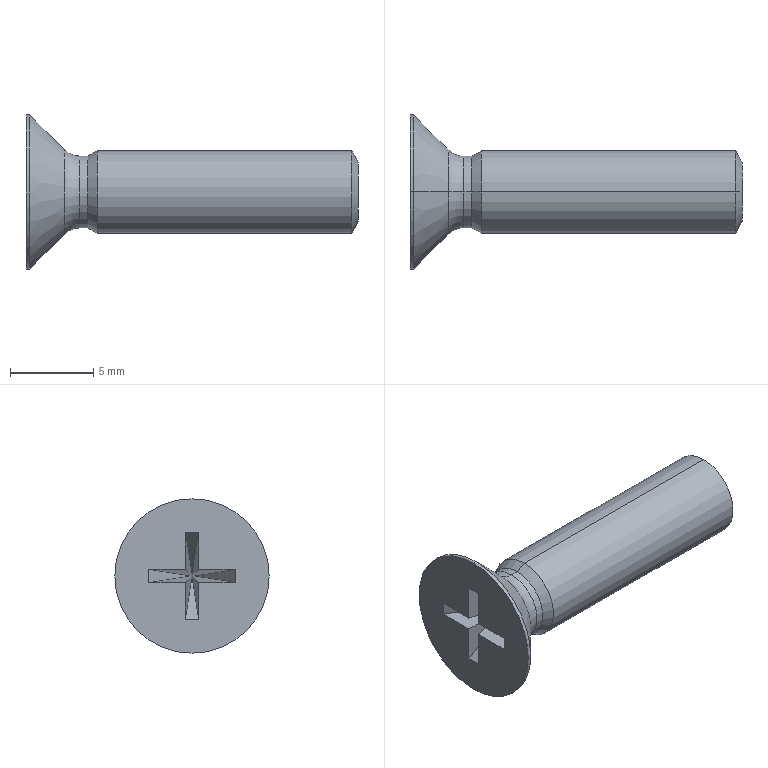Component | SolidWorks | GB_T819.1-2000PhillipsCountersunkHeadScrewM5_20-1 | 1 solid | 28 faces | box 20 x 9.3 x 9.3 mm | volume 433 mm3 | plane 14 | cone 6 | cylinder 6 | torus 2 | commonest cylinder face diameters 5 x2 4.33 x2 9.3 x2
build123d program:
from build123d import *

# Parameters (mm, degrees)
CIRPATTERN1_COUNT = 2
CIRPATTERN1_ANGLE = 90


with BuildPart() as part:
    # Sketch1 → Base-Revolve (revolve)
    with BuildSketch(Plane.XY, mode=Mode.PRIVATE) as base_revolve_sk:
        with BuildLine():
            Line((0, 0), (0, 4.65))
            Line((0, 4.65), (0.215, 4.65))
            Line((0.215, 4.65), (2.319, 2.546))
            ThreePointArc((2.319, 2.546), (2.741, 2.264), (3.238, 2.165))
            Line((3.238, 2.165), (3.72, 2.165))
            Line((3.72, 2.165), (4.3, 2.5))
            Line((4.3, 2.5), (20, 2.5))
            Line((20, 2.5), (20, 0))
            Line((20, 0), (0, 0))
        make_face()
    revolve(base_revolve_sk.sketch.rotate(Axis((0, 0, 0), (1, 0, 0)), 90), axis=Axis((0, 0, 0), (1, 0, 0)))

    # Sketch2 → Cut-Revolve1 (revolve, cut)
    with BuildSketch(Plane.XY, mode=Mode.PRIVATE) as cut_revolve1_sk:
        Polygon((19.604, 2.5), (20.404, 2.5), (20, 1.807), align=None)
    revolve(cut_revolve1_sk.sketch.rotate(Axis((0, 0, 0), (-1, 0, 0)), 270), axis=Axis((0, 0, 0), (-1, 0, 0)), mode=Mode.SUBTRACT)

    # Sketch3 → Cut-Loft1 section 0
    with BuildSketch(Plane.ZY, mode=Mode.PRIVATE) as cut_loft1_s0:
        with BuildLine():
            Line((-2.6, 0.4), (2.6, 0.4))
            Line((2.6, 0.4), (2.6, -0.4))
            Line((2.6, -0.4), (-2.6, -0.4))
            Line((-2.6, -0.4), (-2.6, 0.4))
        make_face()
    cut_loft1 = loft([cut_loft1_s0.sketch, Vertex(3.2, 0, 0)], mode=Mode.SUBTRACT)

    # CirPattern1: Cut-Loft1 ×2 about axis
    cirpattern1_axis = Axis((0, 0, 0), (1, 0, 0))
    for i in range(1, CIRPATTERN1_COUNT):
        add(cut_loft1.rotate(cirpattern1_axis, i * CIRPATTERN1_ANGLE / (CIRPATTERN1_COUNT - 1)), mode=Mode.SUBTRACT)


solid = part.part

# Placed as in the assembly
solid = solid.moved(Location((-247.293, 27.796, 284.382), (0, 0, 0)))